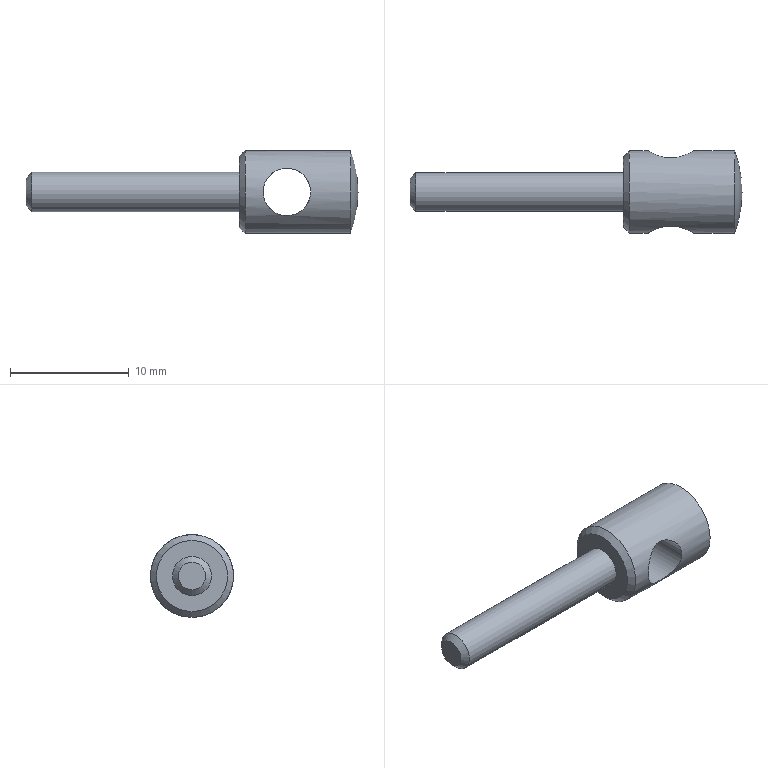Component | NX | 4_GAUGE_CLAMP_PIN | 1 solid | 8 faces | volume 439 mm3 | cylinder 3 | plane 2 | cone 2 | sphere 1 | commonest cylinder face diameters 7 x1 3.3 x1 4 x1